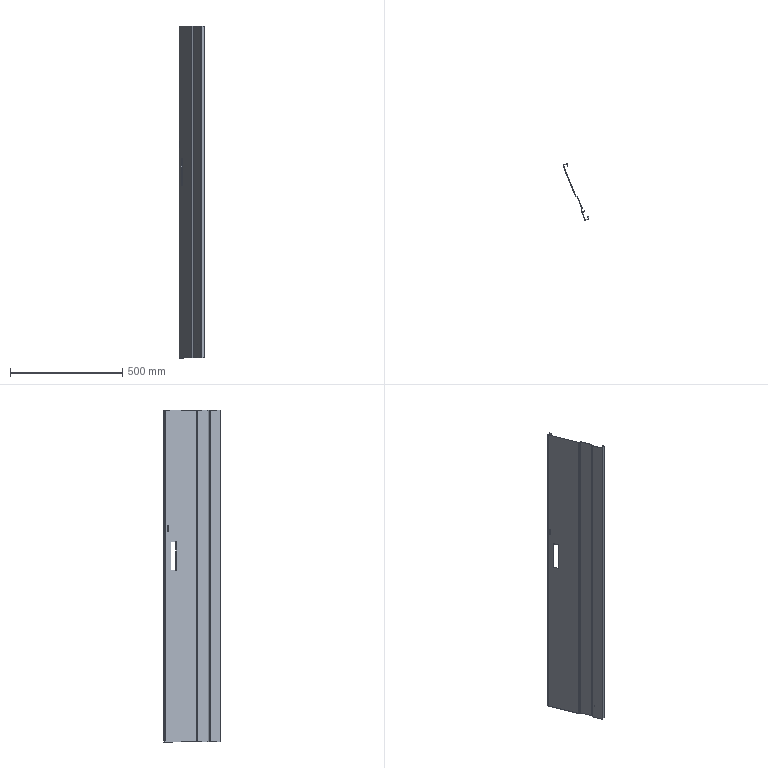Component | SolidWorks | RightDoorAssembly-1_RightDoor-1 | 1 solid | 81 faces | volume 703256 mm3 | plane 63 | cylinder 18 | commonest cylinder face diameters 5 x8 2 x8 4.1 x2